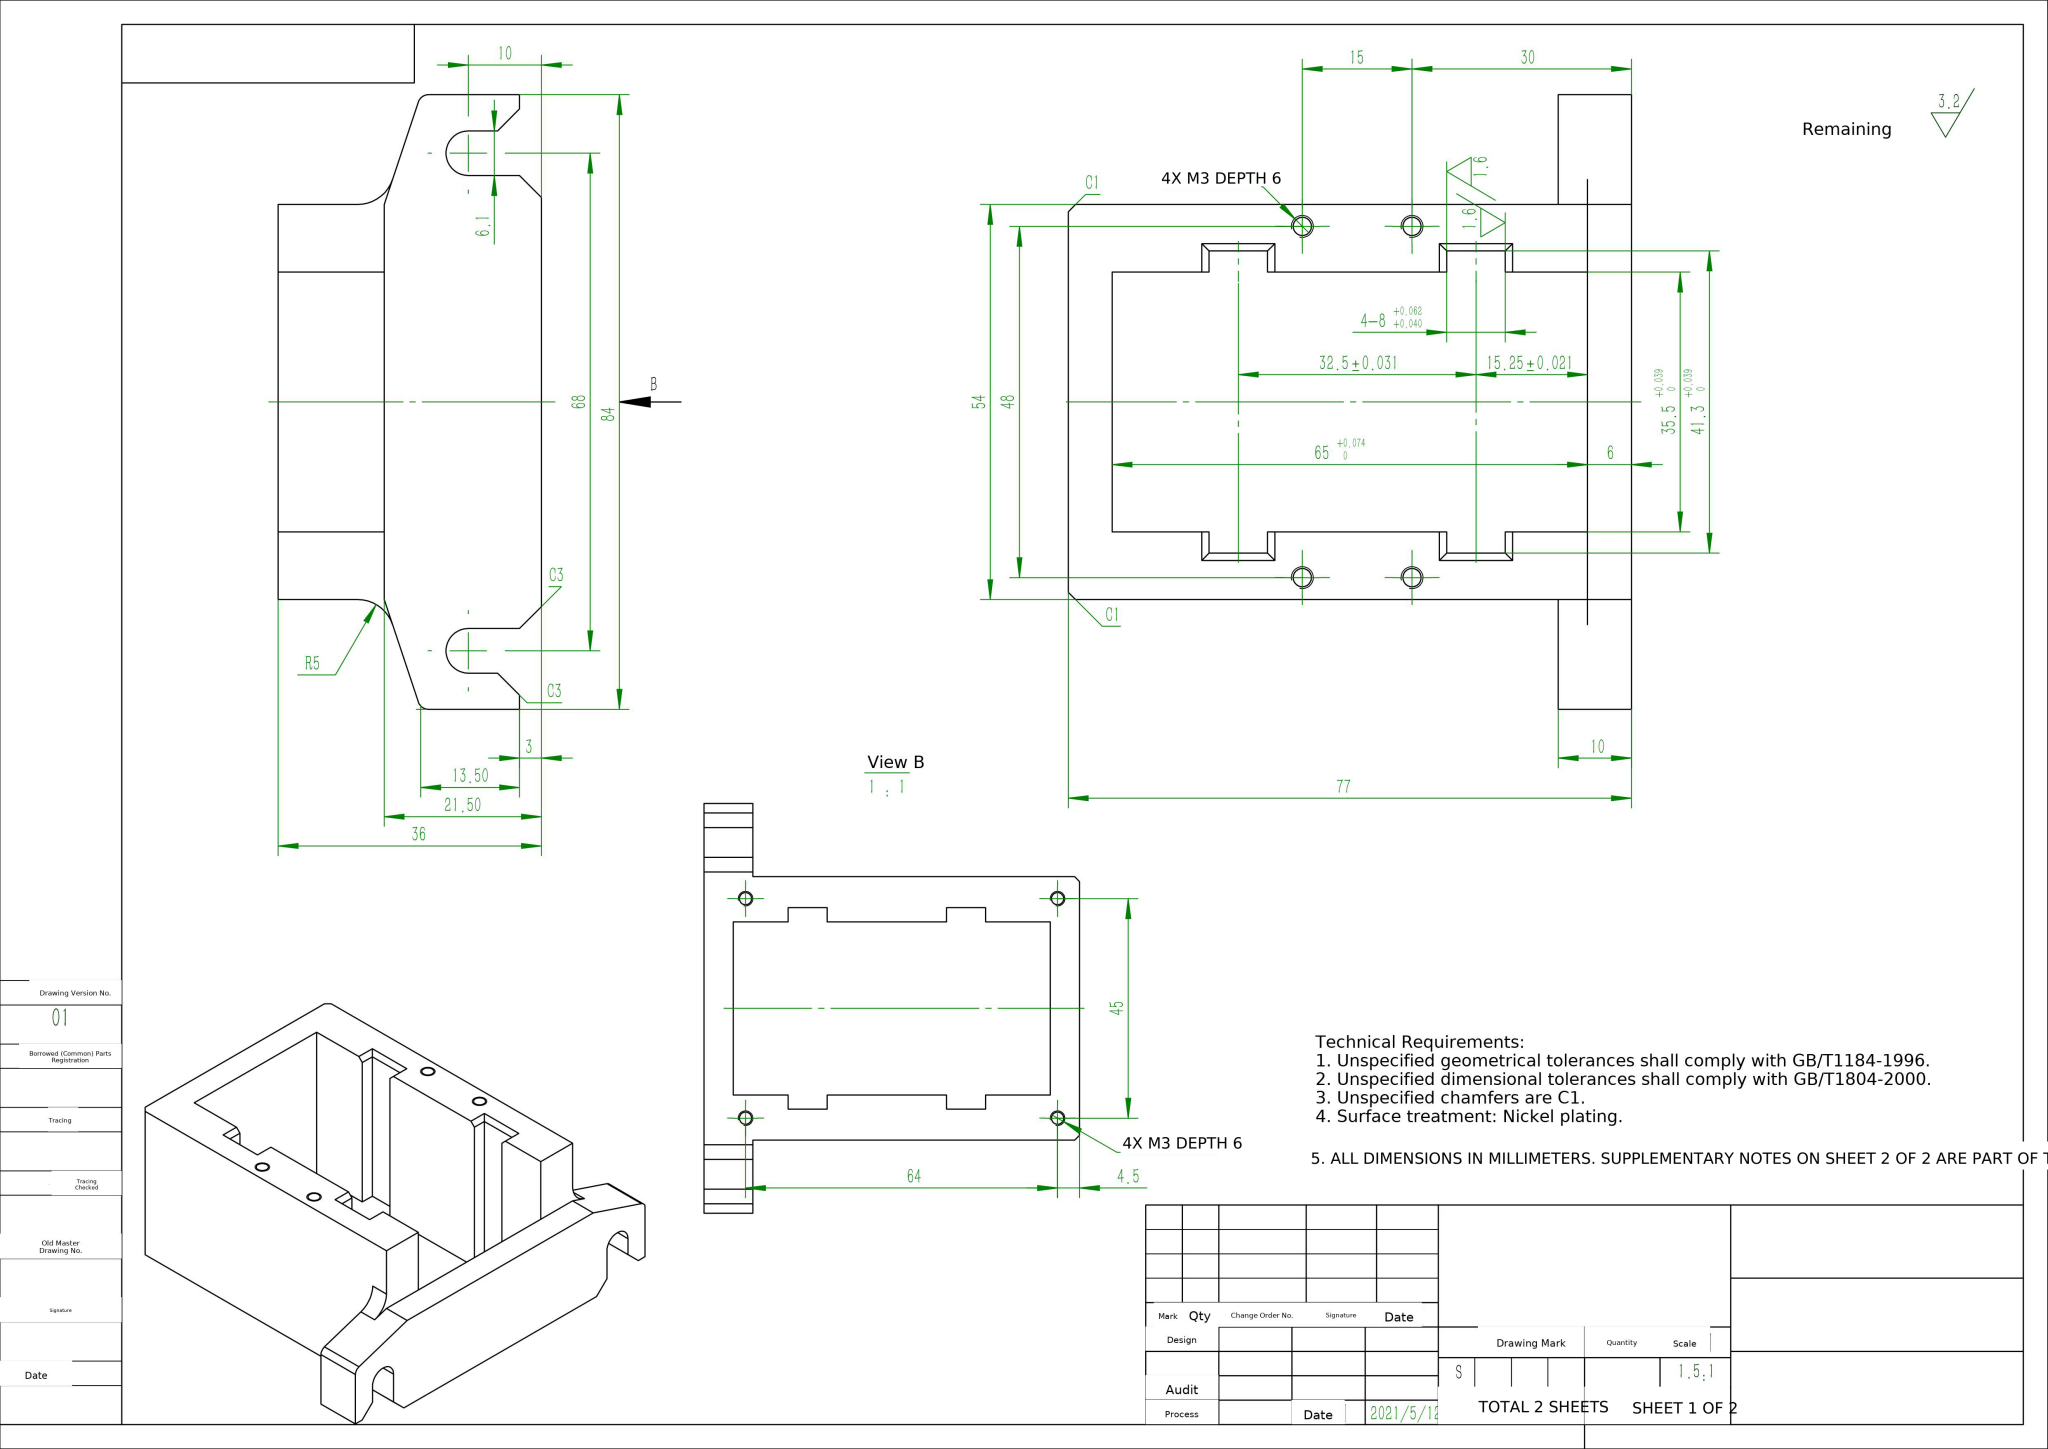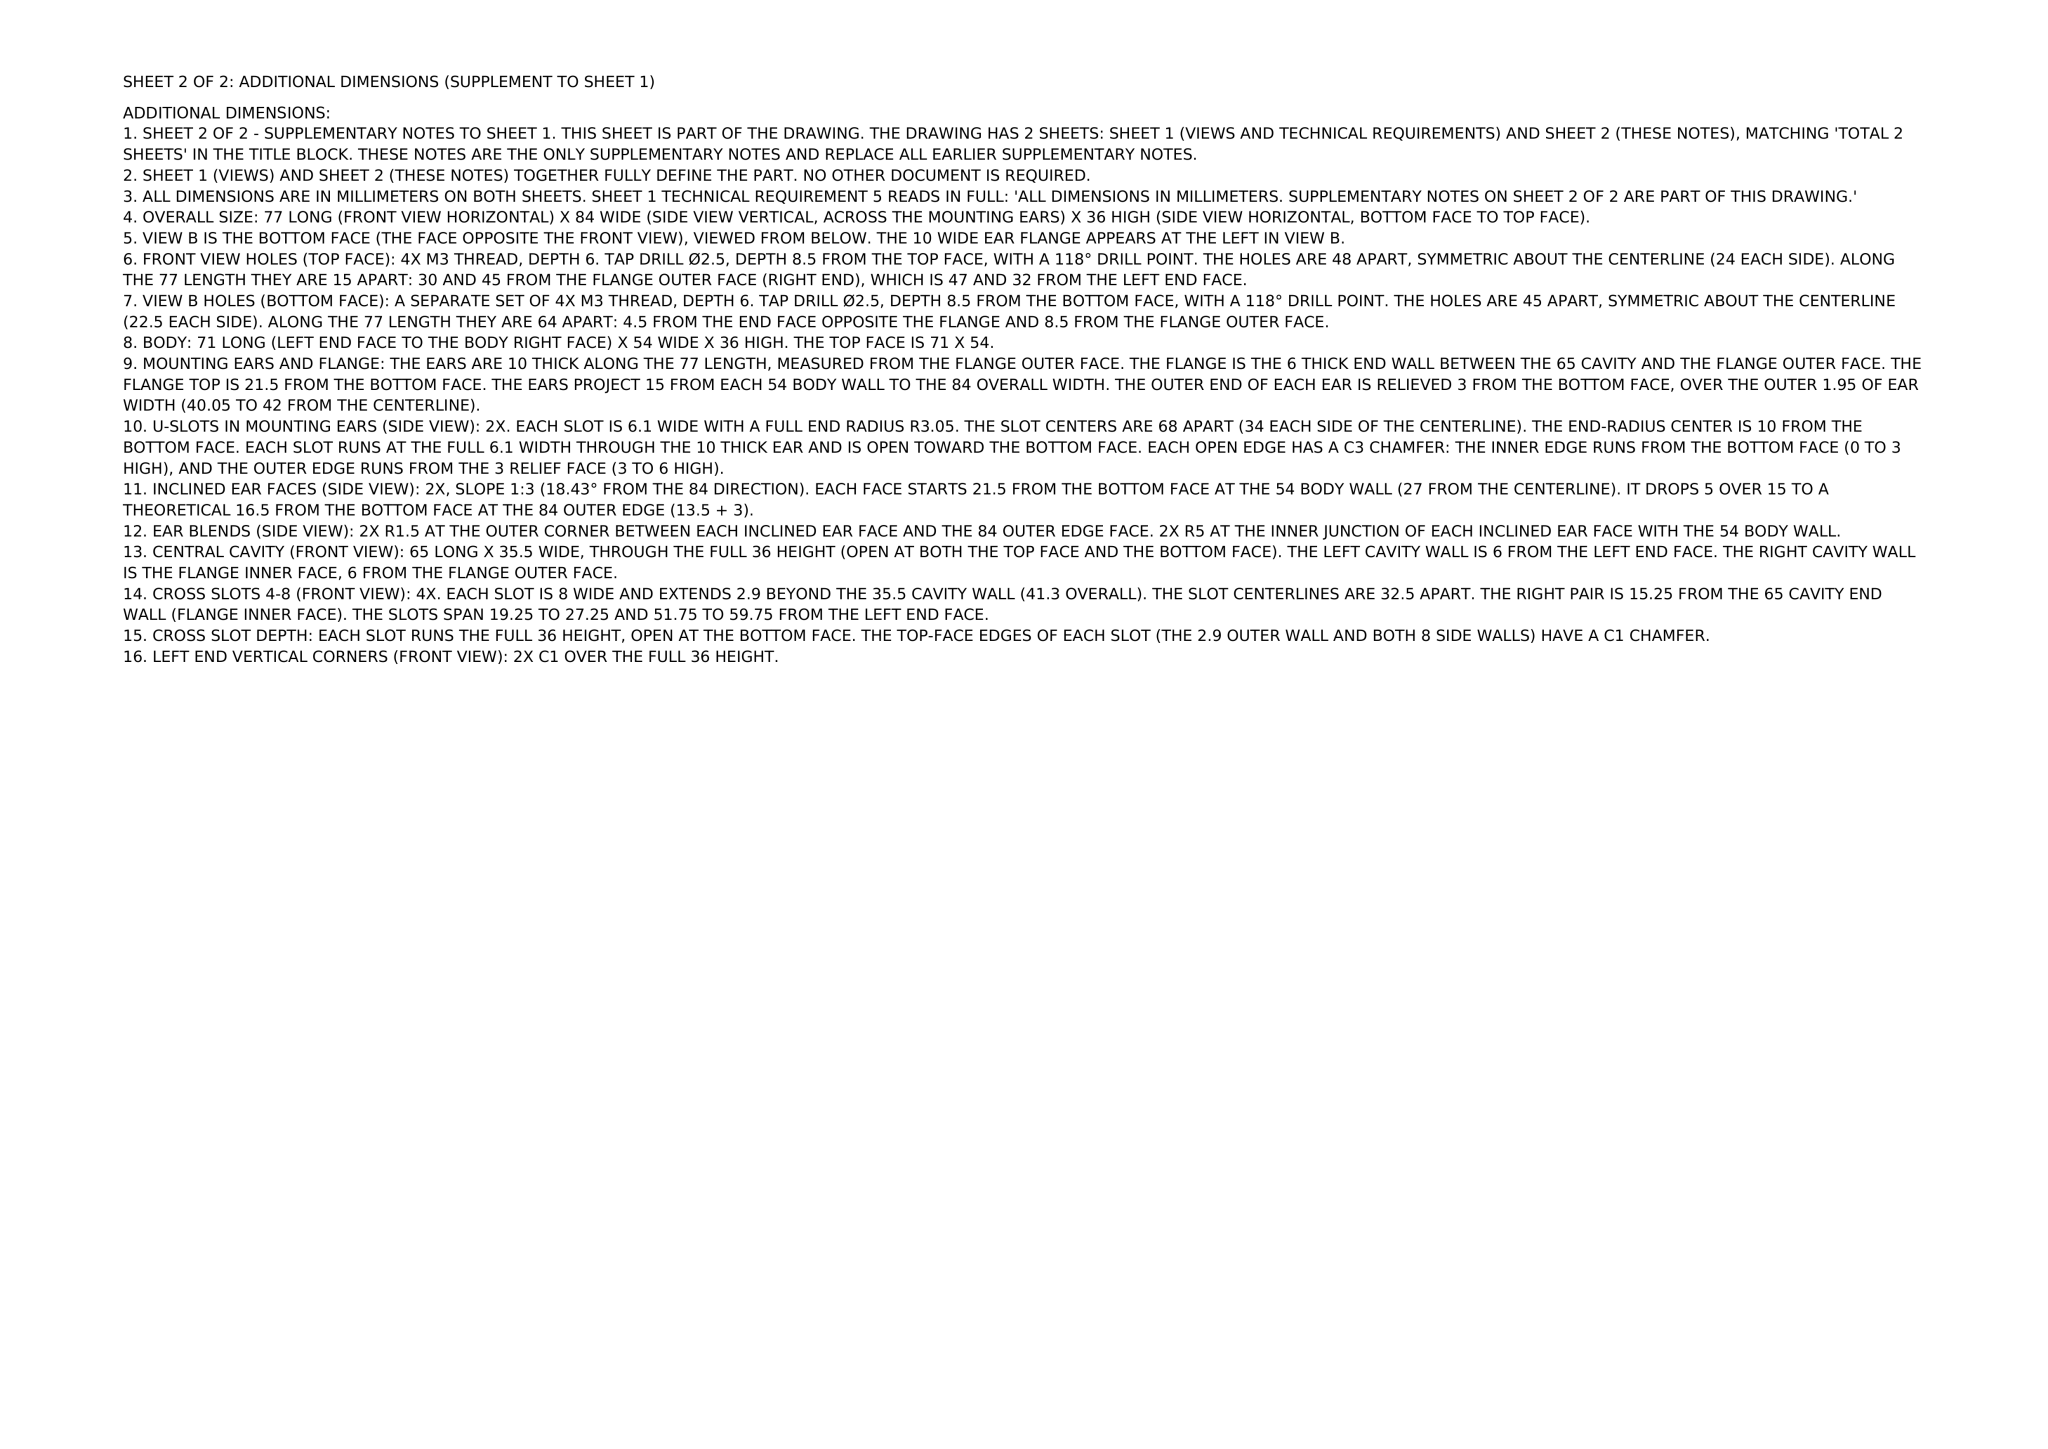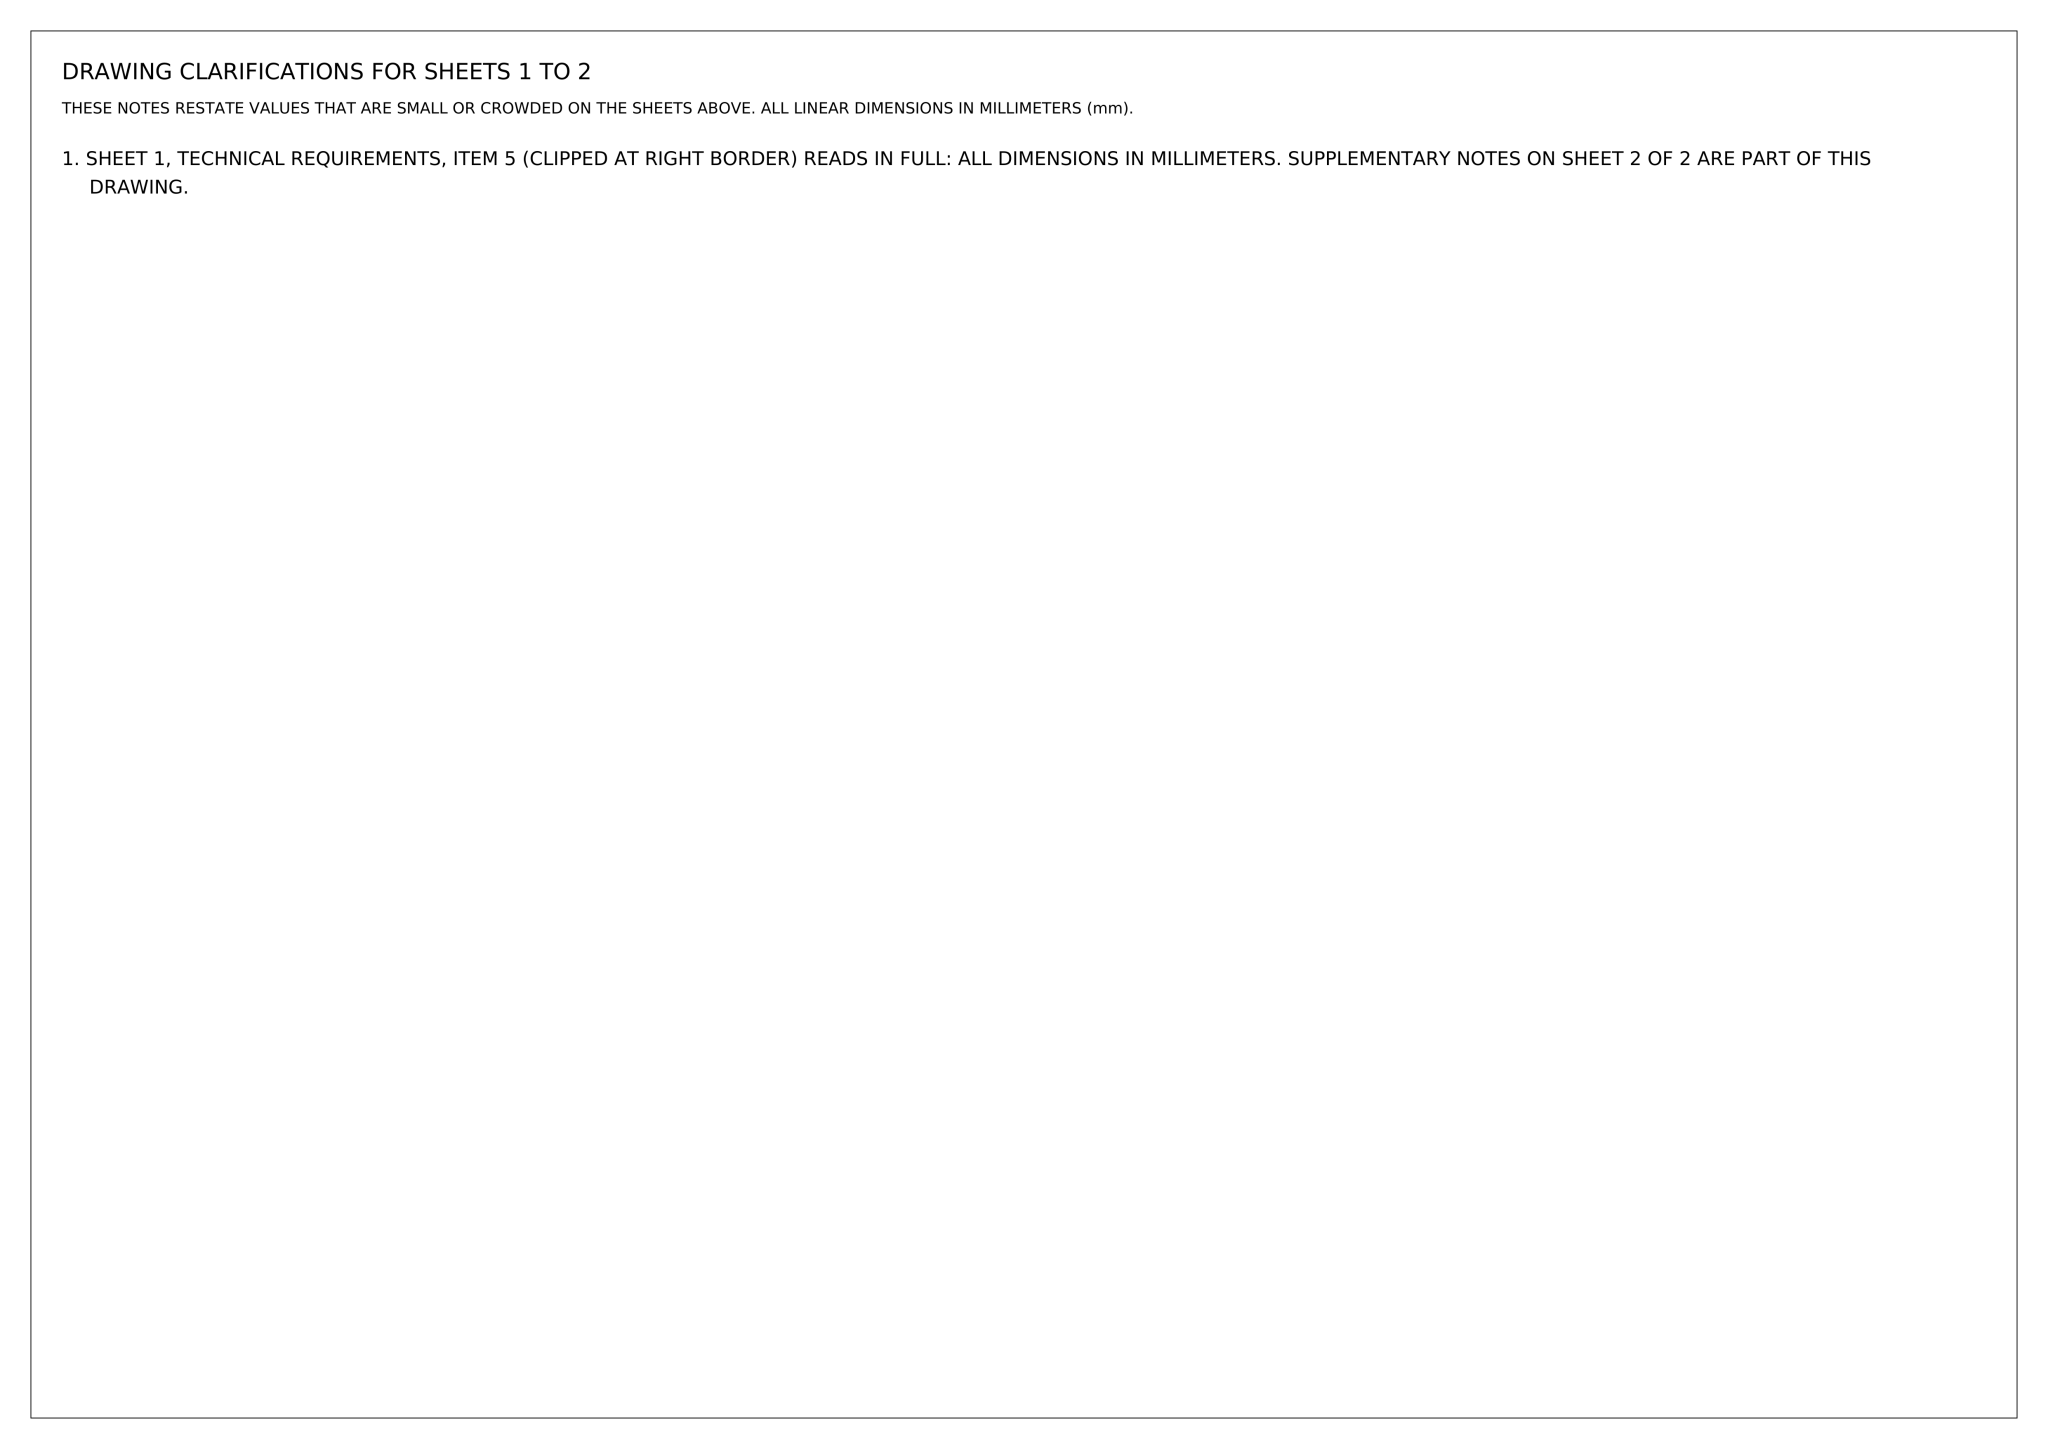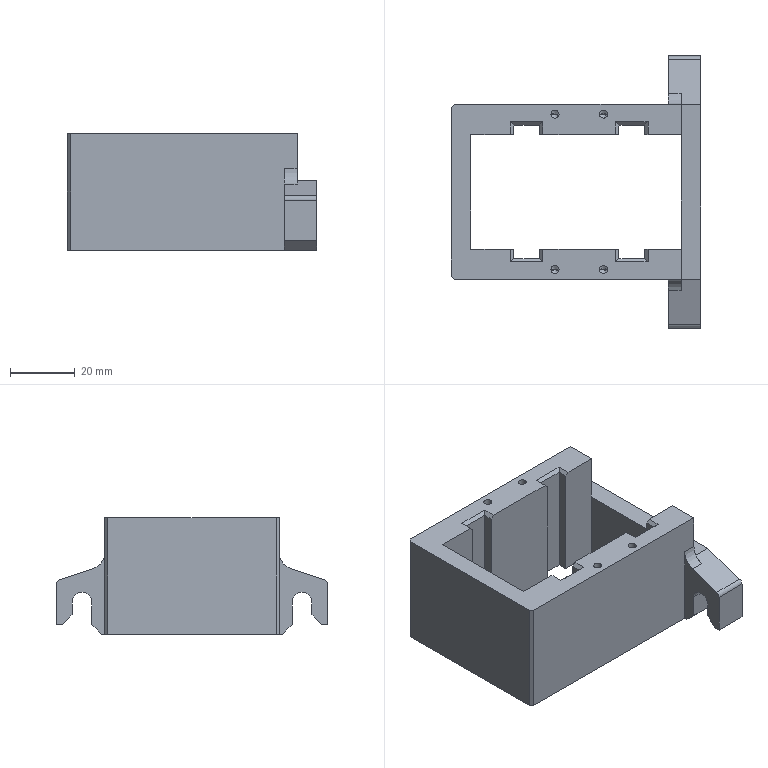Part | NX | mm | 1 solid | 99 faces | box 77 x 84 x 36 mm | volume 61895 mm3 | plane 59 | cylinder 24 | cone 16 | commonest cylinder face diameters 2.5 x16 6.1 x4 10 x2 3 x2